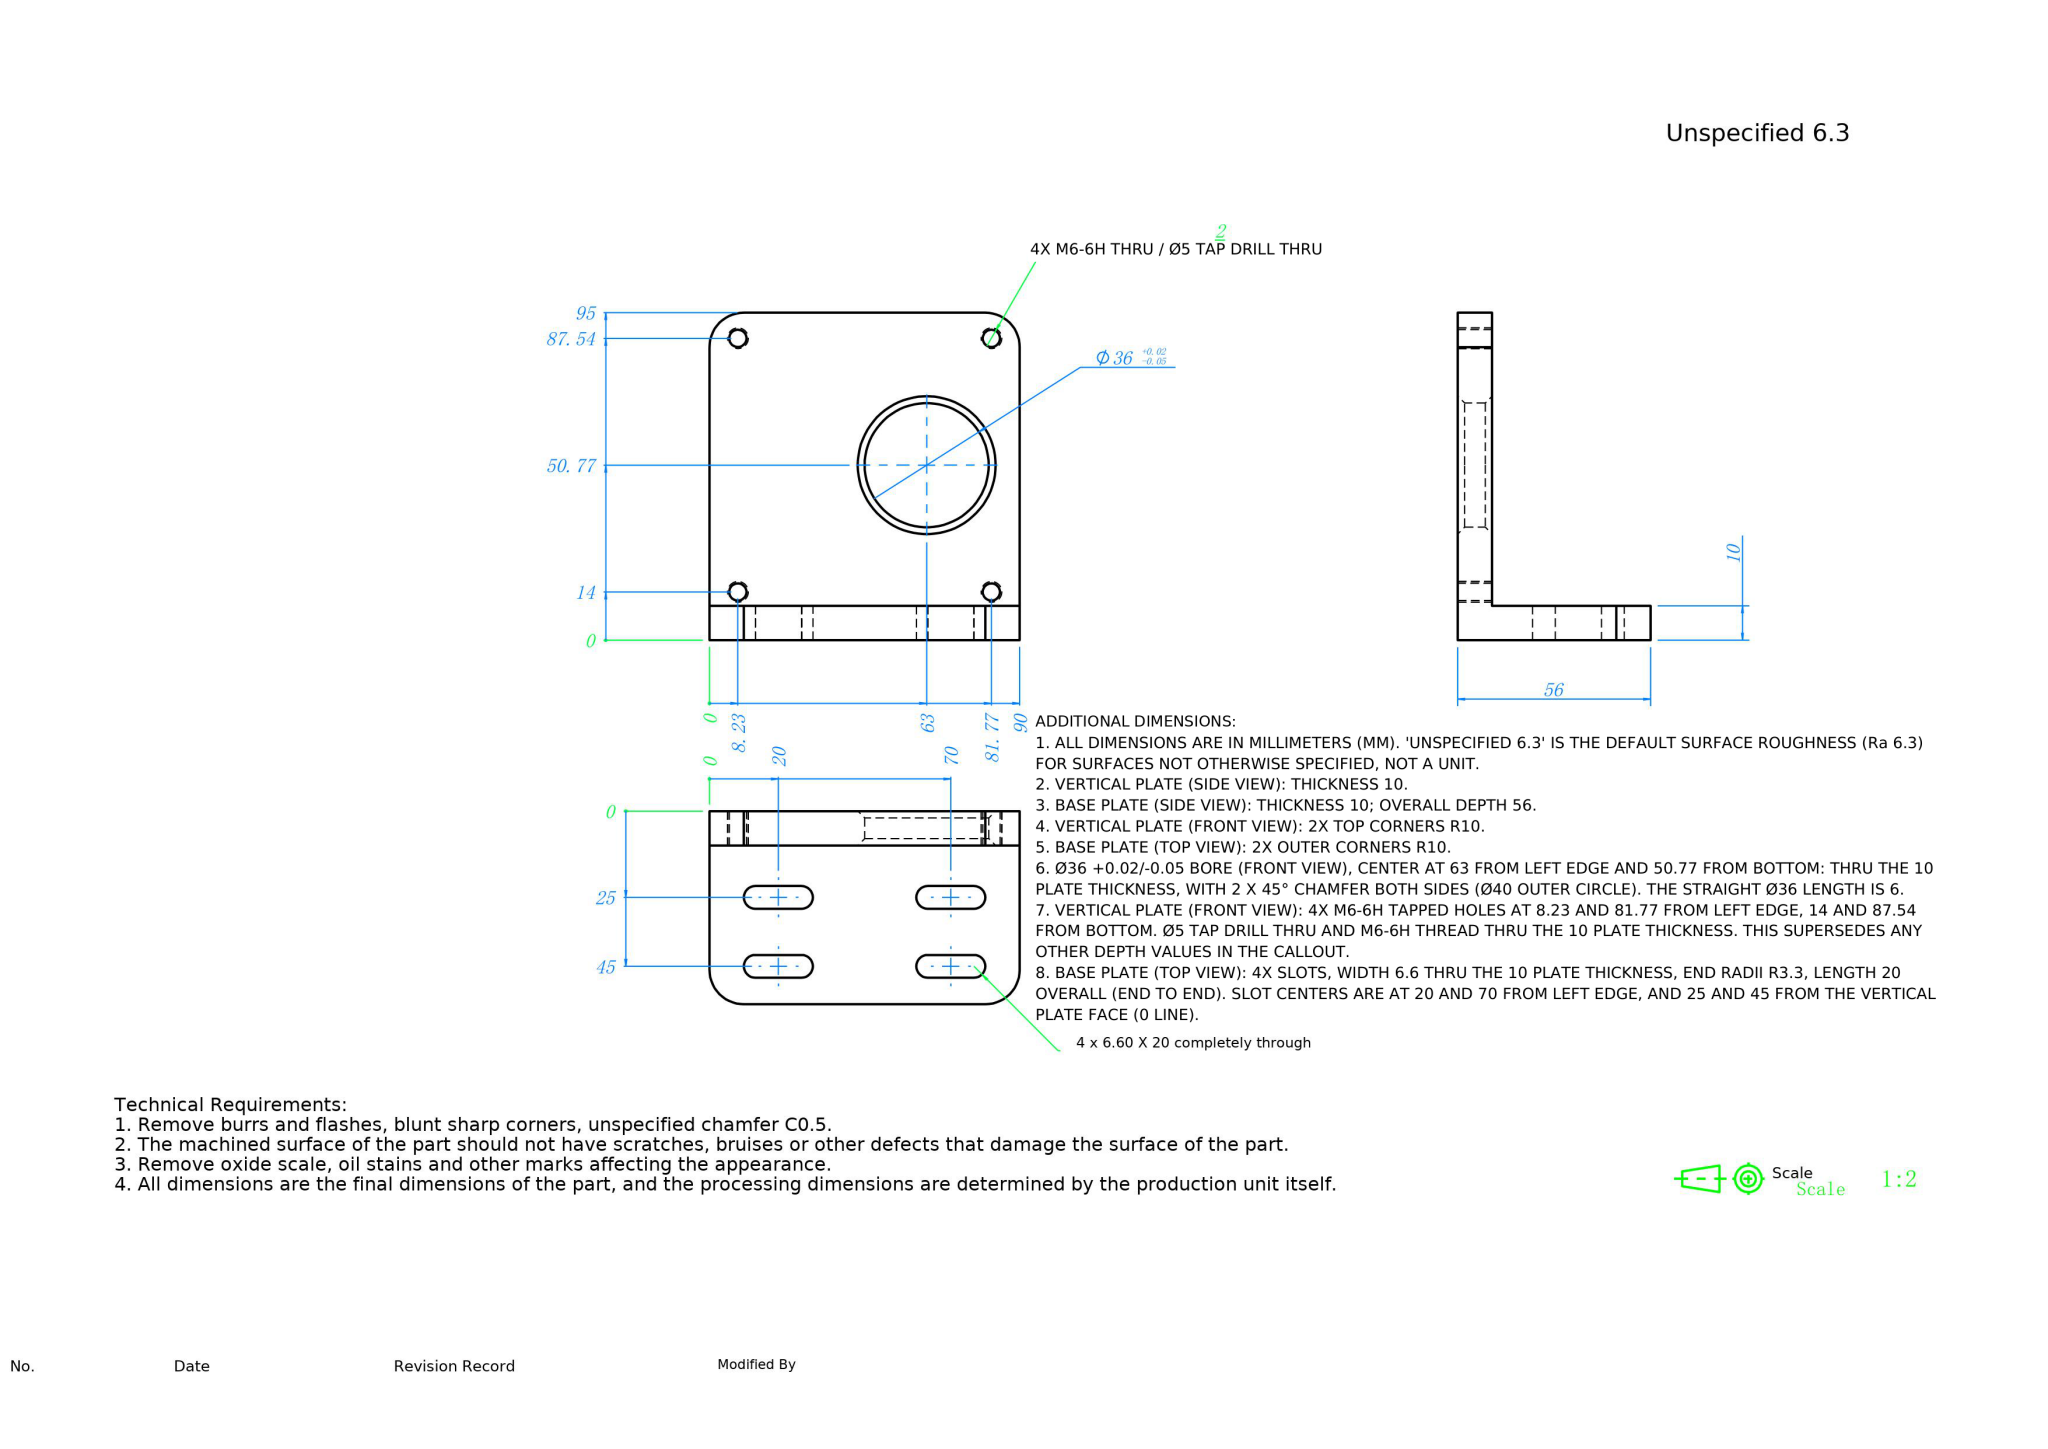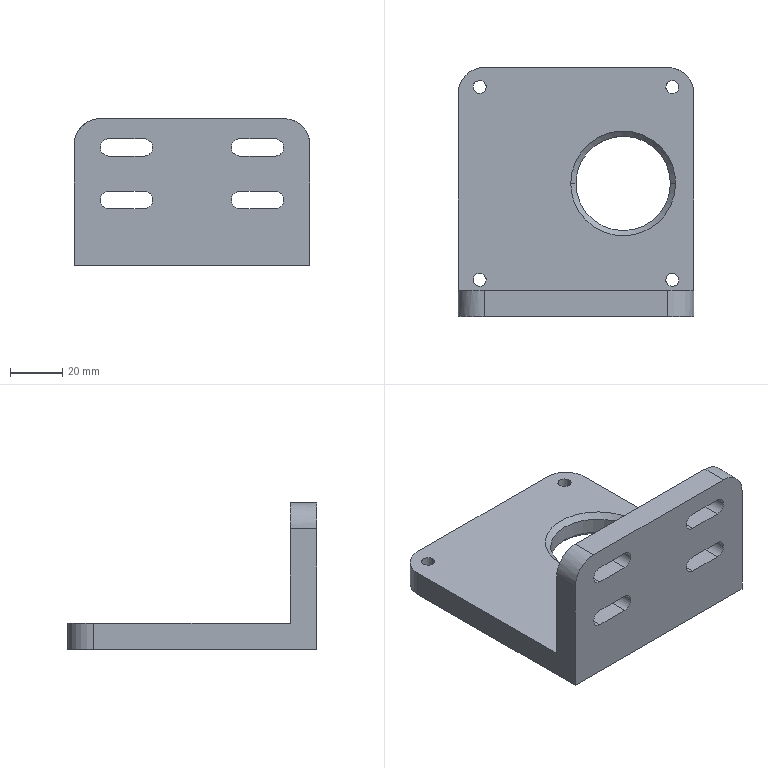Part | NX | mm | 1 solid | 42 faces | box 90 x 95 x 56 mm | volume 109703 mm3 | cylinder 22 | plane 16 | cone 4 | commonest cylinder face diameters 5 x8 6.6 x8 20 x4 36 x2